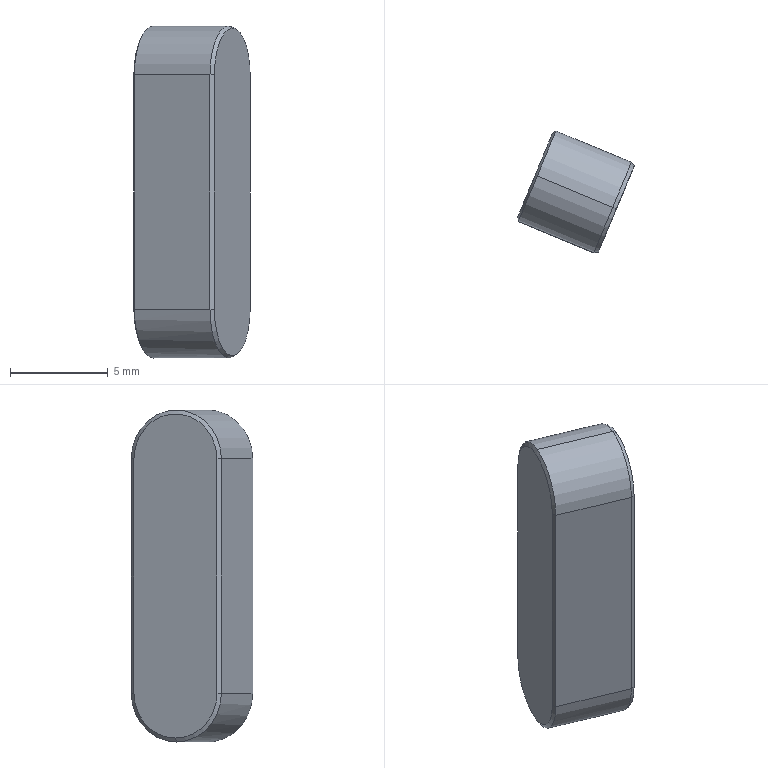Component | SolidWorks | 170423A4-ConveyorSynchronousPulleyAssembly-1_170423A4-Key5x12-1 | 1 solid | 17 faces | box 5.95 x 6.22 x 17 mm | volume 357 mm3 | plane 8 | cone 6 | cylinder 3 | commonest cylinder face diameters 5 x3
build123d program:
from build123d import *
from OCP.BRepFilletAPI import BRepFilletAPI_MakeChamfer

# Parameters (mm, degrees)
BOSS_EXTRUDE1_DEPTH = 4.5
CHAMFER1_SIZE       = 0.2
CHAMFER1_SIZE2      = 0.1155


with BuildPart() as part:
    # Sketch1 → Boss-Extrude1 (new body)
    with BuildSketch(Plane.XY):
        with BuildLine():
            Line((-6, 2.5), (6, 2.5))
            ThreePointArc((6, 2.5), (8.5, 0), (6, -2.5))
            Line((6, -2.5), (-6, -2.5))
            ThreePointArc((-6, -2.5), (-8.5, 0), (-6, 2.5))
        make_face()
    extrude(amount=BOSS_EXTRUDE1_DEPTH)

    # Chamfer1: one chamfer whose edges measure the first distance from different faces: ONE call of the kernel's chamfer builder (chamfer() names one face for all edges)
    chamfer1_edges_1 = [part.edges().sort_by_distance(p)[0] for p in [
        (8.5, 0, 4.5),
    ]]
    chamfer1_side_1 = [part.faces().sort_by_distance(p)[0] for p in [
        (8.5, 0, 2.25),
    ]]
    chamfer1_edges_2 = [part.edges().sort_by_distance(p)[0] for p in [
        (0, 2.5, 4.5),
    ]]
    chamfer1_side_2 = [part.faces().sort_by_distance(p)[0] for p in [
        (0, 2.5, 2.25),
    ]]
    chamfer1_edges_3 = [part.edges().sort_by_distance(p)[0] for p in [
        (-8.5, 0, 4.5),
    ]]
    chamfer1_side_3 = [part.faces().sort_by_distance(p)[0] for p in [
        (-8.5, 0, 2.25),
    ]]
    chamfer1_edges_4 = [part.edges().sort_by_distance(p)[0] for p in [
        (0, 2.5, 0),
        (8.5, 0, 0),
        (0, -2.5, 0),
        (-8.5, 0, 0),
    ]]
    chamfer1_side_4 = [part.faces().sort_by_distance(p)[0] for p in [
        (0, 0, 0),
    ]]
    chamfer1_edges_5 = [part.edges().sort_by_distance(p)[0] for p in [
        (0, -2.5, 4.5),
    ]]
    chamfer1_side_5 = [part.faces().sort_by_distance(p)[0] for p in [
        (0, -2.5, 2.25),
    ]]
    chamfer1 = BRepFilletAPI_MakeChamfer(part.part.solid().wrapped)
    for e in chamfer1_edges_1:
        chamfer1.Add(CHAMFER1_SIZE, CHAMFER1_SIZE2, e.wrapped, chamfer1_side_1[0].wrapped)  # the first distance lies on this face
    for e in chamfer1_edges_2:
        chamfer1.Add(CHAMFER1_SIZE, CHAMFER1_SIZE2, e.wrapped, chamfer1_side_2[0].wrapped)  # the first distance lies on this face
    for e in chamfer1_edges_3:
        chamfer1.Add(CHAMFER1_SIZE, CHAMFER1_SIZE2, e.wrapped, chamfer1_side_3[0].wrapped)  # the first distance lies on this face
    for e in chamfer1_edges_4:
        chamfer1.Add(CHAMFER1_SIZE, CHAMFER1_SIZE2, e.wrapped, chamfer1_side_4[0].wrapped)  # the first distance lies on this face
    for e in chamfer1_edges_5:
        chamfer1.Add(CHAMFER1_SIZE, CHAMFER1_SIZE2, e.wrapped, chamfer1_side_5[0].wrapped)  # the first distance lies on this face
    add(Compound.cast(chamfer1.Shape()), mode=Mode.REPLACE)


solid = part.part

# Placed as in the assembly
solid = solid.moved(Location((103.91, -122.512, 373.3), (90, 67.477, 90)))
STEP:
#1=COLOUR_RGB('',0.7922,0.8196,0.9333);
#2=FILL_AREA_STYLE_COLOUR('',#1);
#3=FILL_AREA_STYLE('',(#2));
#4=SURFACE_STYLE_FILL_AREA(#3);
#5=SURFACE_SIDE_STYLE('',(#4));
#6=SURFACE_STYLE_USAGE(.BOTH.,#5);
#7=PRESENTATION_STYLE_ASSIGNMENT((#6));
#8=CARTESIAN_POINT('',(4.255,-4.891,15.027));
#9=VERTEX_POINT('',#8);
#10=CARTESIAN_POINT('',(4.219,-4.978,14.933));
#11=VERTEX_POINT('',#10);
#12=CARTESIAN_POINT('',(4.255,-4.891,14.933));
#13=DIRECTION('',(0.9237,-0.383,-0.));
#14=DIRECTION('',(0.,0.,-1.));
#15=AXIS2_PLACEMENT_3D('',#12,#13,#14);
#16=CIRCLE('',#15,0.09388);
#17=EDGE_CURVE('',#9,#11,#16,.T.);
#18=ORIENTED_EDGE('',*,*,#17,.F.);
#19=CARTESIAN_POINT('',(4.247,-4.888,15.031));
#20=VERTEX_POINT('',#19);
#21=CARTESIAN_POINT('',(4.255,-4.891,15.027));
#22=DIRECTION('',(-0.8,0.3317,0.5));
#23=VECTOR('',#22,39.37);
#24=LINE('',#21,#23);
#25=EDGE_CURVE('',#9,#20,#24,.T.);
#26=ORIENTED_EDGE('',*,*,#25,.T.);
#27=CARTESIAN_POINT('',(4.21,-4.979,14.933));
#28=VERTEX_POINT('',#27);
#29=CARTESIAN_POINT('',(4.247,-4.888,14.933));
#30=DIRECTION('',(-0.9237,0.383,0.));
#31=DIRECTION('',(0.,0.,-1.));
#32=AXIS2_PLACEMENT_3D('',#29,#30,#31);
#33=CIRCLE('',#32,0.09843);
#34=EDGE_CURVE('',#28,#20,#33,.T.);
#35=ORIENTED_EDGE('',*,*,#34,.F.);
#36=CARTESIAN_POINT('',(4.21,-4.979,14.933));
#37=DIRECTION('',(0.9915,0.1301,0.));
#38=VECTOR('',#37,39.37);
#39=LINE('',#36,#38);
#40=EDGE_CURVE('',#28,#11,#39,.T.);
#41=ORIENTED_EDGE('',*,*,#40,.T.);
#42=EDGE_LOOP('',(#18,#26,#35,#41));
#43=FACE_OUTER_BOUND('',#42,.T.);
#44=CARTESIAN_POINT('',(4.255,-4.891,14.933));
#45=DIRECTION('',(-0.9237,0.383,0.));
#46=DIRECTION('',(0.,-0.,1.));
#47=AXIS2_PLACEMENT_3D('',#44,#45,#46);
#48=CONICAL_SURFACE('',#47,0.09388,0.5236);
#49=ADVANCED_FACE('',(#43),#48,.T.);
#50=CARTESIAN_POINT('',(4.091,-4.823,14.37));
#51=VERTEX_POINT('',#50);
#52=CARTESIAN_POINT('',(4.056,-4.907,14.461));
#53=VERTEX_POINT('',#52);
#54=CARTESIAN_POINT('',(4.091,-4.823,14.461));
#55=DIRECTION('',(-0.9237,0.383,0.));
#56=DIRECTION('',(0.,0.,-1.));
#57=AXIS2_PLACEMENT_3D('',#54,#55,#56);
#58=CIRCLE('',#57,0.09055);
#59=EDGE_CURVE('',#51,#53,#58,.T.);
#60=ORIENTED_EDGE('',*,*,#59,.F.);
#61=CARTESIAN_POINT('',(4.095,-4.825,14.362));
#62=VERTEX_POINT('',#61);
#63=CARTESIAN_POINT('',(4.095,-4.825,14.362));
#64=DIRECTION('',(0.4619,-0.1915,-0.866));
#65=VECTOR('',#64,39.37);
#66=LINE('',#63,#65);
#67=EDGE_CURVE('',#51,#62,#66,.T.);
#68=ORIENTED_EDGE('',*,*,#67,.T.);
#69=CARTESIAN_POINT('',(4.057,-4.916,14.461));
#70=VERTEX_POINT('',#69);
#71=CARTESIAN_POINT('',(4.095,-4.825,14.461));
#72=DIRECTION('',(0.9237,-0.383,-0.));
#73=DIRECTION('',(0.,0.,-1.));
#74=AXIS2_PLACEMENT_3D('',#71,#72,#73);
#75=CIRCLE('',#74,0.09843);
#76=EDGE_CURVE('',#70,#62,#75,.T.);
#77=ORIENTED_EDGE('',*,*,#76,.F.);
#78=CARTESIAN_POINT('',(4.056,-4.907,14.461));
#79=DIRECTION('',(0.1301,-0.9915,-0.));
#80=VECTOR('',#79,39.37);
#81=LINE('',#78,#80);
#82=EDGE_CURVE('',#53,#70,#81,.T.);
#83=ORIENTED_EDGE('',*,*,#82,.F.);
#84=EDGE_LOOP('',(#60,#68,#77,#83));
#85=FACE_OUTER_BOUND('',#84,.T.);
#86=CARTESIAN_POINT('',(4.095,-4.825,14.461));
#87=DIRECTION('',(0.9237,-0.383,-0.));
#88=DIRECTION('',(0.,0.,-1.));
#89=AXIS2_PLACEMENT_3D('',#86,#87,#88);
#90=CONICAL_SURFACE('',#89,0.09843,1.047);
#91=ADVANCED_FACE('',(#85),#90,.T.);
#92=ORIENTED_EDGE('',*,*,#34,.T.);
#93=CARTESIAN_POINT('',(4.095,-4.825,15.031));
#94=VERTEX_POINT('',#93);
#95=CARTESIAN_POINT('',(4.255,-4.891,15.031));
#96=DIRECTION('',(-0.9237,0.383,0.));
#97=VECTOR('',#96,39.37);
#98=LINE('',#95,#97);
#99=EDGE_CURVE('',#20,#94,#98,.T.);
#100=ORIENTED_EDGE('',*,*,#99,.T.);
#101=CARTESIAN_POINT('',(4.057,-4.916,14.933));
#102=VERTEX_POINT('',#101);
#103=CARTESIAN_POINT('',(4.095,-4.825,14.933));
#104=DIRECTION('',(0.9237,-0.383,-0.));
#105=DIRECTION('',(0.,0.,-1.));
#106=AXIS2_PLACEMENT_3D('',#103,#104,#105);
#107=CIRCLE('',#106,0.09843);
#108=EDGE_CURVE('',#94,#102,#107,.T.);
#109=ORIENTED_EDGE('',*,*,#108,.T.);
#110=CARTESIAN_POINT('',(4.217,-4.982,14.933));
#111=DIRECTION('',(-0.9237,0.383,0.));
#112=VECTOR('',#111,39.37);
#113=LINE('',#110,#112);
#114=EDGE_CURVE('',#28,#102,#113,.T.);
#115=ORIENTED_EDGE('',*,*,#114,.F.);
#116=EDGE_LOOP('',(#92,#100,#109,#115));
#117=FACE_OUTER_BOUND('',#116,.T.);
#118=CARTESIAN_POINT('',(4.255,-4.891,14.933));
#119=DIRECTION('',(-0.9237,0.383,0.));
#120=DIRECTION('',(0.,-0.,1.));
#121=AXIS2_PLACEMENT_3D('',#118,#119,#120);
#122=CYLINDRICAL_SURFACE('',#121,0.09843);
#123=ADVANCED_FACE('',(#117),#122,.T.);
#124=ORIENTED_EDGE('',*,*,#99,.F.);
#125=CARTESIAN_POINT('',(4.285,-4.797,14.933));
#126=VERTEX_POINT('',#125);
#127=CARTESIAN_POINT('',(4.247,-4.888,14.933));
#128=DIRECTION('',(-0.9237,0.383,0.));
#129=DIRECTION('',(0.,0.,-1.));
#130=AXIS2_PLACEMENT_3D('',#127,#128,#129);
#131=CIRCLE('',#130,0.09843);
#132=EDGE_CURVE('',#20,#126,#131,.T.);
#133=ORIENTED_EDGE('',*,*,#132,.T.);
#134=CARTESIAN_POINT('',(4.133,-4.734,14.933));
#135=VERTEX_POINT('',#134);
#136=CARTESIAN_POINT('',(4.292,-4.8,14.933));
#137=DIRECTION('',(-0.9237,0.383,0.));
#138=VECTOR('',#137,39.37);
#139=LINE('',#136,#138);
#140=EDGE_CURVE('',#126,#135,#139,.T.);
#141=ORIENTED_EDGE('',*,*,#140,.T.);
#142=CARTESIAN_POINT('',(4.095,-4.825,14.933));
#143=DIRECTION('',(0.9237,-0.383,-0.));
#144=DIRECTION('',(0.,0.,-1.));
#145=AXIS2_PLACEMENT_3D('',#142,#143,#144);
#146=CIRCLE('',#145,0.09843);
#147=EDGE_CURVE('',#135,#94,#146,.T.);
#148=ORIENTED_EDGE('',*,*,#147,.T.);
#149=EDGE_LOOP('',(#124,#133,#141,#148));
#150=FACE_OUTER_BOUND('',#149,.T.);
#151=CARTESIAN_POINT('',(4.255,-4.891,14.933));
#152=DIRECTION('',(-0.9237,0.383,0.));
#153=DIRECTION('',(0.,-0.,1.));
#154=AXIS2_PLACEMENT_3D('',#151,#152,#153);
#155=CYLINDRICAL_SURFACE('',#154,0.09843);
#156=ADVANCED_FACE('',(#150),#155,.T.);
#157=ORIENTED_EDGE('',*,*,#114,.T.);
#158=CARTESIAN_POINT('',(4.057,-4.916,14.933));
#159=DIRECTION('',(-0.,0.,-1.));
#160=VECTOR('',#159,39.37);
#161=LINE('',#158,#160);
#162=EDGE_CURVE('',#102,#70,#161,.T.);
#163=ORIENTED_EDGE('',*,*,#162,.T.);
#164=CARTESIAN_POINT('',(4.21,-4.979,14.461));
#165=VERTEX_POINT('',#164);
#166=CARTESIAN_POINT('',(4.217,-4.982,14.461));
#167=DIRECTION('',(-0.9237,0.383,0.));
#168=VECTOR('',#167,39.37);
#169=LINE('',#166,#168);
#170=EDGE_CURVE('',#165,#70,#169,.T.);
#171=ORIENTED_EDGE('',*,*,#170,.F.);
#172=CARTESIAN_POINT('',(4.21,-4.979,14.933));
#173=DIRECTION('',(0.,-0.,1.));
#174=VECTOR('',#173,39.37);
#175=LINE('',#172,#174);
#176=EDGE_CURVE('',#165,#28,#175,.T.);
#177=ORIENTED_EDGE('',*,*,#176,.T.);
#178=EDGE_LOOP('',(#157,#163,#171,#177));
#179=FACE_OUTER_BOUND('',#178,.T.);
#180=CARTESIAN_POINT('',(4.217,-4.982,14.933));
#181=DIRECTION('',(0.383,0.9237,0.));
#182=DIRECTION('',(0.9237,-0.383,-0.));
#183=AXIS2_PLACEMENT_3D('',#180,#181,#182);
#184=PLANE('',#183);
#185=ADVANCED_FACE('',(#179),#184,.F.);
#186=ORIENTED_EDGE('',*,*,#170,.T.);
#187=ORIENTED_EDGE('',*,*,#76,.T.);
#188=CARTESIAN_POINT('',(4.133,-4.734,14.461));
#189=VERTEX_POINT('',#188);
#190=CARTESIAN_POINT('',(4.095,-4.825,14.461));
#191=DIRECTION('',(0.9237,-0.383,-0.));
#192=DIRECTION('',(0.,0.,-1.));
#193=AXIS2_PLACEMENT_3D('',#190,#191,#192);
#194=CIRCLE('',#193,0.09843);
#195=EDGE_CURVE('',#62,#189,#194,.T.);
#196=ORIENTED_EDGE('',*,*,#195,.T.);
#197=CARTESIAN_POINT('',(4.285,-4.797,14.461));
#198=VERTEX_POINT('',#197);
#199=CARTESIAN_POINT('',(4.292,-4.8,14.461));
#200=DIRECTION('',(-0.9237,0.383,0.));
#201=VECTOR('',#200,39.37);
#202=LINE('',#199,#201);
#203=EDGE_CURVE('',#198,#189,#202,.T.);
#204=ORIENTED_EDGE('',*,*,#203,.F.);
#205=CARTESIAN_POINT('',(4.247,-4.888,14.461));
#206=DIRECTION('',(-0.9237,0.383,0.));
#207=DIRECTION('',(0.,0.,-1.));
#208=AXIS2_PLACEMENT_3D('',#205,#206,#207);
#209=CIRCLE('',#208,0.09843);
#210=EDGE_CURVE('',#198,#165,#209,.T.);
#211=ORIENTED_EDGE('',*,*,#210,.T.);
#212=EDGE_LOOP('',(#186,#187,#196,#204,#211));
#213=FACE_OUTER_BOUND('',#212,.T.);
#214=CARTESIAN_POINT('',(4.255,-4.891,14.461));
#215=DIRECTION('',(-0.9237,0.383,0.));
#216=DIRECTION('',(0.,-0.,1.));
#217=AXIS2_PLACEMENT_3D('',#214,#215,#216);
#218=CYLINDRICAL_SURFACE('',#217,0.09843);
#219=ADVANCED_FACE('',(#213),#218,.T.);
#220=ORIENTED_EDGE('',*,*,#203,.T.);
#221=CARTESIAN_POINT('',(4.133,-4.734,14.933));
#222=DIRECTION('',(0.,-0.,1.));
#223=VECTOR('',#222,39.37);
#224=LINE('',#221,#223);
#225=EDGE_CURVE('',#189,#135,#224,.T.);
#226=ORIENTED_EDGE('',*,*,#225,.T.);
#227=ORIENTED_EDGE('',*,*,#140,.F.);
#228=CARTESIAN_POINT('',(4.285,-4.797,14.461));
#229=DIRECTION('',(-0.,0.,-1.));
#230=VECTOR('',#229,39.37);
#231=LINE('',#228,#230);
#232=EDGE_CURVE('',#126,#198,#231,.T.);
#233=ORIENTED_EDGE('',*,*,#232,.T.);
#234=EDGE_LOOP('',(#220,#226,#227,#233));
#235=FACE_OUTER_BOUND('',#234,.T.);
#236=CARTESIAN_POINT('',(4.292,-4.8,14.933));
#237=DIRECTION('',(-0.383,-0.9237,-0.));
#238=DIRECTION('',(-0.,0.,-1.));
#239=AXIS2_PLACEMENT_3D('',#236,#237,#238);
#240=PLANE('',#239);
#241=ADVANCED_FACE('',(#235),#240,.F.);
#242=CARTESIAN_POINT('',(4.219,-4.978,14.461));
#243=VERTEX_POINT('',#242);
#244=CARTESIAN_POINT('',(4.291,-4.804,14.461));
#245=VERTEX_POINT('',#244);
#246=CARTESIAN_POINT('',(4.255,-4.891,14.461));
#247=DIRECTION('',(0.9237,-0.383,-0.));
#248=DIRECTION('',(0.,0.,-1.));
#249=AXIS2_PLACEMENT_3D('',#246,#247,#248);
#250=CIRCLE('',#249,0.09388);
#251=EDGE_CURVE('',#243,#245,#250,.T.);
#252=ORIENTED_EDGE('',*,*,#251,.T.);
#253=CARTESIAN_POINT('',(4.291,-4.804,14.933));
#254=VERTEX_POINT('',#253);
#255=CARTESIAN_POINT('',(4.291,-4.804,14.933));
#256=DIRECTION('',(0.,-0.,1.));
#257=VECTOR('',#256,39.37);
#258=LINE('',#255,#257);
#259=EDGE_CURVE('',#245,#254,#258,.T.);
#260=ORIENTED_EDGE('',*,*,#259,.T.);
#261=CARTESIAN_POINT('',(4.255,-4.891,14.933));
#262=DIRECTION('',(0.9237,-0.383,-0.));
#263=DIRECTION('',(0.,0.,-1.));
#264=AXIS2_PLACEMENT_3D('',#261,#262,#263);
#265=CIRCLE('',#264,0.09388);
#266=EDGE_CURVE('',#254,#9,#265,.T.);
#267=ORIENTED_EDGE('',*,*,#266,.T.);
#268=ORIENTED_EDGE('',*,*,#17,.T.);
#269=CARTESIAN_POINT('',(4.219,-4.978,14.461));
#270=DIRECTION('',(-0.,0.,-1.));
#271=VECTOR('',#270,39.37);
#272=LINE('',#269,#271);
#273=EDGE_CURVE('',#11,#243,#272,.T.);
#274=ORIENTED_EDGE('',*,*,#273,.T.);
#275=EDGE_LOOP('',(#252,#260,#267,#268,#274));
#276=FACE_OUTER_BOUND('',#275,.T.);
#277=CARTESIAN_POINT('',(4.255,-4.891,14.933));
#278=DIRECTION('',(0.9237,-0.383,-0.));
#279=DIRECTION('',(-0.,0.,-1.));
#280=AXIS2_PLACEMENT_3D('',#277,#278,#279);
#281=PLANE('',#280);
#282=ADVANCED_FACE('',(#276),#281,.T.);
#283=CARTESIAN_POINT('',(4.126,-4.74,14.461));
#284=VERTEX_POINT('',#283);
#285=CARTESIAN_POINT('',(4.091,-4.823,14.461));
#286=DIRECTION('',(-0.9237,0.383,0.));
#287=DIRECTION('',(0.,0.,-1.));
#288=AXIS2_PLACEMENT_3D('',#285,#286,#287);
#289=CIRCLE('',#288,0.09055);
#290=EDGE_CURVE('',#284,#51,#289,.T.);
#291=ORIENTED_EDGE('',*,*,#290,.T.);
#292=ORIENTED_EDGE('',*,*,#59,.T.);
#293=CARTESIAN_POINT('',(4.056,-4.907,14.933));
#294=VERTEX_POINT('',#293);
#295=CARTESIAN_POINT('',(4.056,-4.907,14.933));
#296=DIRECTION('',(0.,-0.,1.));
#297=VECTOR('',#296,39.37);
#298=LINE('',#295,#297);
#299=EDGE_CURVE('',#53,#294,#298,.T.);
#300=ORIENTED_EDGE('',*,*,#299,.T.);
#301=CARTESIAN_POINT('',(4.126,-4.74,14.933));
#302=VERTEX_POINT('',#301);
#303=CARTESIAN_POINT('',(4.091,-4.823,14.933));
#304=DIRECTION('',(-0.9237,0.383,0.));
#305=DIRECTION('',(0.,0.,-1.));
#306=AXIS2_PLACEMENT_3D('',#303,#304,#305);
#307=CIRCLE('',#306,0.09055);
#308=EDGE_CURVE('',#294,#302,#307,.T.);
#309=ORIENTED_EDGE('',*,*,#308,.T.);
#310=CARTESIAN_POINT('',(4.126,-4.74,14.933));
#311=DIRECTION('',(-0.,0.,-1.));
#312=VECTOR('',#311,39.37);
#313=LINE('',#310,#312);
#314=EDGE_CURVE('',#302,#284,#313,.T.);
#315=ORIENTED_EDGE('',*,*,#314,.T.);
#316=EDGE_LOOP('',(#291,#292,#300,#309,#315));
#317=FACE_OUTER_BOUND('',#316,.T.);
#318=CARTESIAN_POINT('',(4.091,-4.823,14.933));
#319=DIRECTION('',(0.9237,-0.383,-0.));
#320=DIRECTION('',(-0.,0.,-1.));
#321=AXIS2_PLACEMENT_3D('',#318,#319,#320);
#322=PLANE('',#321);
#323=ADVANCED_FACE('',(#317),#322,.F.);
#324=CARTESIAN_POINT('',(4.126,-4.74,14.461));
#325=DIRECTION('',(0.7936,0.6084,0.));
#326=VECTOR('',#325,39.37);
#327=LINE('',#324,#326);
#328=EDGE_CURVE('',#284,#189,#327,.T.);
#329=ORIENTED_EDGE('',*,*,#328,.F.);
#330=ORIENTED_EDGE('',*,*,#314,.F.);
#331=CARTESIAN_POINT('',(4.133,-4.734,14.933));
#332=DIRECTION('',(-0.7936,-0.6084,-0.));
#333=VECTOR('',#332,39.37);
#334=LINE('',#331,#333);
#335=EDGE_CURVE('',#135,#302,#334,.T.);
#336=ORIENTED_EDGE('',*,*,#335,.F.);
#337=ORIENTED_EDGE('',*,*,#225,.F.);
#338=EDGE_LOOP('',(#329,#330,#336,#337));
#339=FACE_OUTER_BOUND('',#338,.T.);
#340=CARTESIAN_POINT('',(4.133,-4.734,14.933));
#341=DIRECTION('',(0.6084,-0.7936,-0.));
#342=DIRECTION('',(0.,-0.,1.));
#343=AXIS2_PLACEMENT_3D('',#340,#341,#342);
#344=PLANE('',#343);
#345=ADVANCED_FACE('',(#339),#344,.F.);
#346=ORIENTED_EDGE('',*,*,#335,.T.);
#347=ORIENTED_EDGE('',*,*,#308,.F.);
#348=CARTESIAN_POINT('',(4.057,-4.916,14.933));
#349=DIRECTION('',(-0.1301,0.9915,0.));
#350=VECTOR('',#349,39.37);
#351=LINE('',#348,#350);
#352=EDGE_CURVE('',#102,#294,#351,.T.);
#353=ORIENTED_EDGE('',*,*,#352,.F.);
#354=ORIENTED_EDGE('',*,*,#108,.F.);
#355=ORIENTED_EDGE('',*,*,#147,.F.);
#356=EDGE_LOOP('',(#346,#347,#353,#354,#355));
#357=FACE_OUTER_BOUND('',#356,.T.);
#358=CARTESIAN_POINT('',(4.095,-4.825,14.933));
#359=DIRECTION('',(0.9237,-0.383,-0.));
#360=DIRECTION('',(0.,0.,-1.));
#361=AXIS2_PLACEMENT_3D('',#358,#359,#360);
#362=CONICAL_SURFACE('',#361,0.09843,1.047);
#363=ADVANCED_FACE('',(#357),#362,.T.);
#364=ORIENTED_EDGE('',*,*,#67,.F.);
#365=ORIENTED_EDGE('',*,*,#290,.F.);
#366=ORIENTED_EDGE('',*,*,#328,.T.);
#367=ORIENTED_EDGE('',*,*,#195,.F.);
#368=EDGE_LOOP('',(#364,#365,#366,#367));
#369=FACE_OUTER_BOUND('',#368,.T.);
#370=CARTESIAN_POINT('',(4.095,-4.825,14.461));
#371=DIRECTION('',(0.9237,-0.383,-0.));
#372=DIRECTION('',(0.,0.,-1.));
#373=AXIS2_PLACEMENT_3D('',#370,#371,#372);
#374=CONICAL_SURFACE('',#373,0.09843,1.047);
#375=ADVANCED_FACE('',(#369),#374,.T.);
#376=ORIENTED_EDGE('',*,*,#352,.T.);
#377=ORIENTED_EDGE('',*,*,#299,.F.);
#378=ORIENTED_EDGE('',*,*,#82,.T.);
#379=ORIENTED_EDGE('',*,*,#162,.F.);
#380=EDGE_LOOP('',(#376,#377,#378,#379));
#381=FACE_OUTER_BOUND('',#380,.T.);
#382=CARTESIAN_POINT('',(4.057,-4.916,14.933));
#383=DIRECTION('',(0.9915,0.1301,0.));
#384=DIRECTION('',(-0.,0.,-1.));
#385=AXIS2_PLACEMENT_3D('',#382,#383,#384);
#386=PLANE('',#385);
#387=ADVANCED_FACE('',(#381),#386,.F.);
#388=ORIENTED_EDGE('',*,*,#40,.F.);
#389=ORIENTED_EDGE('',*,*,#176,.F.);
#390=CARTESIAN_POINT('',(4.219,-4.978,14.461));
#391=DIRECTION('',(-0.9915,-0.1301,-0.));
#392=VECTOR('',#391,39.37);
#393=LINE('',#390,#392);
#394=EDGE_CURVE('',#243,#165,#393,.T.);
#395=ORIENTED_EDGE('',*,*,#394,.F.);
#396=ORIENTED_EDGE('',*,*,#273,.F.);
#397=EDGE_LOOP('',(#388,#389,#395,#396));
#398=FACE_OUTER_BOUND('',#397,.T.);
#399=CARTESIAN_POINT('',(4.219,-4.978,14.933));
#400=DIRECTION('',(0.1301,-0.9915,-0.));
#401=DIRECTION('',(0.,-0.,1.));
#402=AXIS2_PLACEMENT_3D('',#399,#400,#401);
#403=PLANE('',#402);
#404=ADVANCED_FACE('',(#398),#403,.T.);
#405=ORIENTED_EDGE('',*,*,#394,.T.);
#406=ORIENTED_EDGE('',*,*,#210,.F.);
#407=CARTESIAN_POINT('',(4.291,-4.804,14.461));
#408=DIRECTION('',(-0.6084,0.7936,0.));
#409=VECTOR('',#408,39.37);
#410=LINE('',#407,#409);
#411=EDGE_CURVE('',#245,#198,#410,.T.);
#412=ORIENTED_EDGE('',*,*,#411,.F.);
#413=ORIENTED_EDGE('',*,*,#251,.F.);
#414=EDGE_LOOP('',(#405,#406,#412,#413));
#415=FACE_OUTER_BOUND('',#414,.T.);
#416=CARTESIAN_POINT('',(4.255,-4.891,14.461));
#417=DIRECTION('',(-0.9237,0.383,0.));
#418=DIRECTION('',(0.,-0.,1.));
#419=AXIS2_PLACEMENT_3D('',#416,#417,#418);
#420=CONICAL_SURFACE('',#419,0.09388,0.5236);
#421=ADVANCED_FACE('',(#415),#420,.T.);
#422=ORIENTED_EDGE('',*,*,#25,.F.);
#423=ORIENTED_EDGE('',*,*,#266,.F.);
#424=CARTESIAN_POINT('',(4.285,-4.797,14.933));
#425=DIRECTION('',(0.6084,-0.7936,-0.));
#426=VECTOR('',#425,39.37);
#427=LINE('',#424,#426);
#428=EDGE_CURVE('',#126,#254,#427,.T.);
#429=ORIENTED_EDGE('',*,*,#428,.F.);
#430=ORIENTED_EDGE('',*,*,#132,.F.);
#431=EDGE_LOOP('',(#422,#423,#429,#430));
#432=FACE_OUTER_BOUND('',#431,.T.);
#433=CARTESIAN_POINT('',(4.255,-4.891,14.933));
#434=DIRECTION('',(-0.9237,0.383,0.));
#435=DIRECTION('',(0.,-0.,1.));
#436=AXIS2_PLACEMENT_3D('',#433,#434,#435);
#437=CONICAL_SURFACE('',#436,0.09388,0.5236);
#438=ADVANCED_FACE('',(#432),#437,.T.);
#439=ORIENTED_EDGE('',*,*,#411,.T.);
#440=ORIENTED_EDGE('',*,*,#232,.F.);
#441=ORIENTED_EDGE('',*,*,#428,.T.);
#442=ORIENTED_EDGE('',*,*,#259,.F.);
#443=EDGE_LOOP('',(#439,#440,#441,#442));
#444=FACE_OUTER_BOUND('',#443,.T.);
#445=CARTESIAN_POINT('',(4.291,-4.804,14.933));
#446=DIRECTION('',(0.7936,0.6084,0.));
#447=DIRECTION('',(-0.,0.,-1.));
#448=AXIS2_PLACEMENT_3D('',#445,#446,#447);
#449=PLANE('',#448);
#450=ADVANCED_FACE('',(#444),#449,.T.);
#451=CLOSED_SHELL('',(#49,#91,#123,#156,#185,#219,#241,#282,#323,#345,#363,#375,#387,#404,#421,#438,#450));
#452=MANIFOLD_SOLID_BREP('',#451);
#453=STYLED_ITEM('',(#7),#452);
#454=(LENGTH_UNIT()NAMED_UNIT(*)SI_UNIT($,.METRE.));
#455=LENGTH_MEASURE_WITH_UNIT(LENGTH_MEASURE(0.0254),#454);
#456=DIMENSIONAL_EXPONENTS(1.,0.,0.,0.,0.,0.,0.);
#457=(CONVERSION_BASED_UNIT('',#455)LENGTH_UNIT()NAMED_UNIT(#456));
#458=UNCERTAINTY_MEASURE_WITH_UNIT(LENGTH_MEASURE(0.00001),#457,'','');
#459=(NAMED_UNIT(*)PLANE_ANGLE_UNIT()SI_UNIT($,.RADIAN.));
#460=(NAMED_UNIT(*)SI_UNIT($,.STERADIAN.)SOLID_ANGLE_UNIT());
#461=(GEOMETRIC_REPRESENTATION_CONTEXT(3)GLOBAL_UNCERTAINTY_ASSIGNED_CONTEXT((#458))GLOBAL_UNIT_ASSIGNED_CONTEXT((#457,#459,#460))REPRESENTATION_CONTEXT('',''));
#462=MECHANICAL_DESIGN_GEOMETRIC_PRESENTATION_REPRESENTATION('',(#453),#461);
#463=CARTESIAN_POINT('',(0.,0.,0.));
#464=DIRECTION('',(0.,0.,1.));
#465=DIRECTION('',(1.,0.,0.));
#466=AXIS2_PLACEMENT_3D('',#463,#464,#465);
#467=(LENGTH_UNIT()NAMED_UNIT(*)SI_UNIT($,.METRE.));
#468=LENGTH_MEASURE_WITH_UNIT(LENGTH_MEASURE(0.0254),#467);
#469=DIMENSIONAL_EXPONENTS(1.,0.,0.,0.,0.,0.,0.);
#470=(CONVERSION_BASED_UNIT('',#468)LENGTH_UNIT()NAMED_UNIT(#469));
#471=UNCERTAINTY_MEASURE_WITH_UNIT(LENGTH_MEASURE(0.00001),#470,'','');
#472=(NAMED_UNIT(*)PLANE_ANGLE_UNIT()SI_UNIT($,.RADIAN.));
#473=(NAMED_UNIT(*)SI_UNIT($,.STERADIAN.)SOLID_ANGLE_UNIT());
#474=(GEOMETRIC_REPRESENTATION_CONTEXT(3)GLOBAL_UNCERTAINTY_ASSIGNED_CONTEXT((#471))GLOBAL_UNIT_ASSIGNED_CONTEXT((#470,#472,#473))REPRESENTATION_CONTEXT('',''));
#475=ADVANCED_BREP_SHAPE_REPRESENTATION('',(#452,#466),#474);
#476=PRESENTATION_LAYER_ASSIGNMENT('','',(#453));